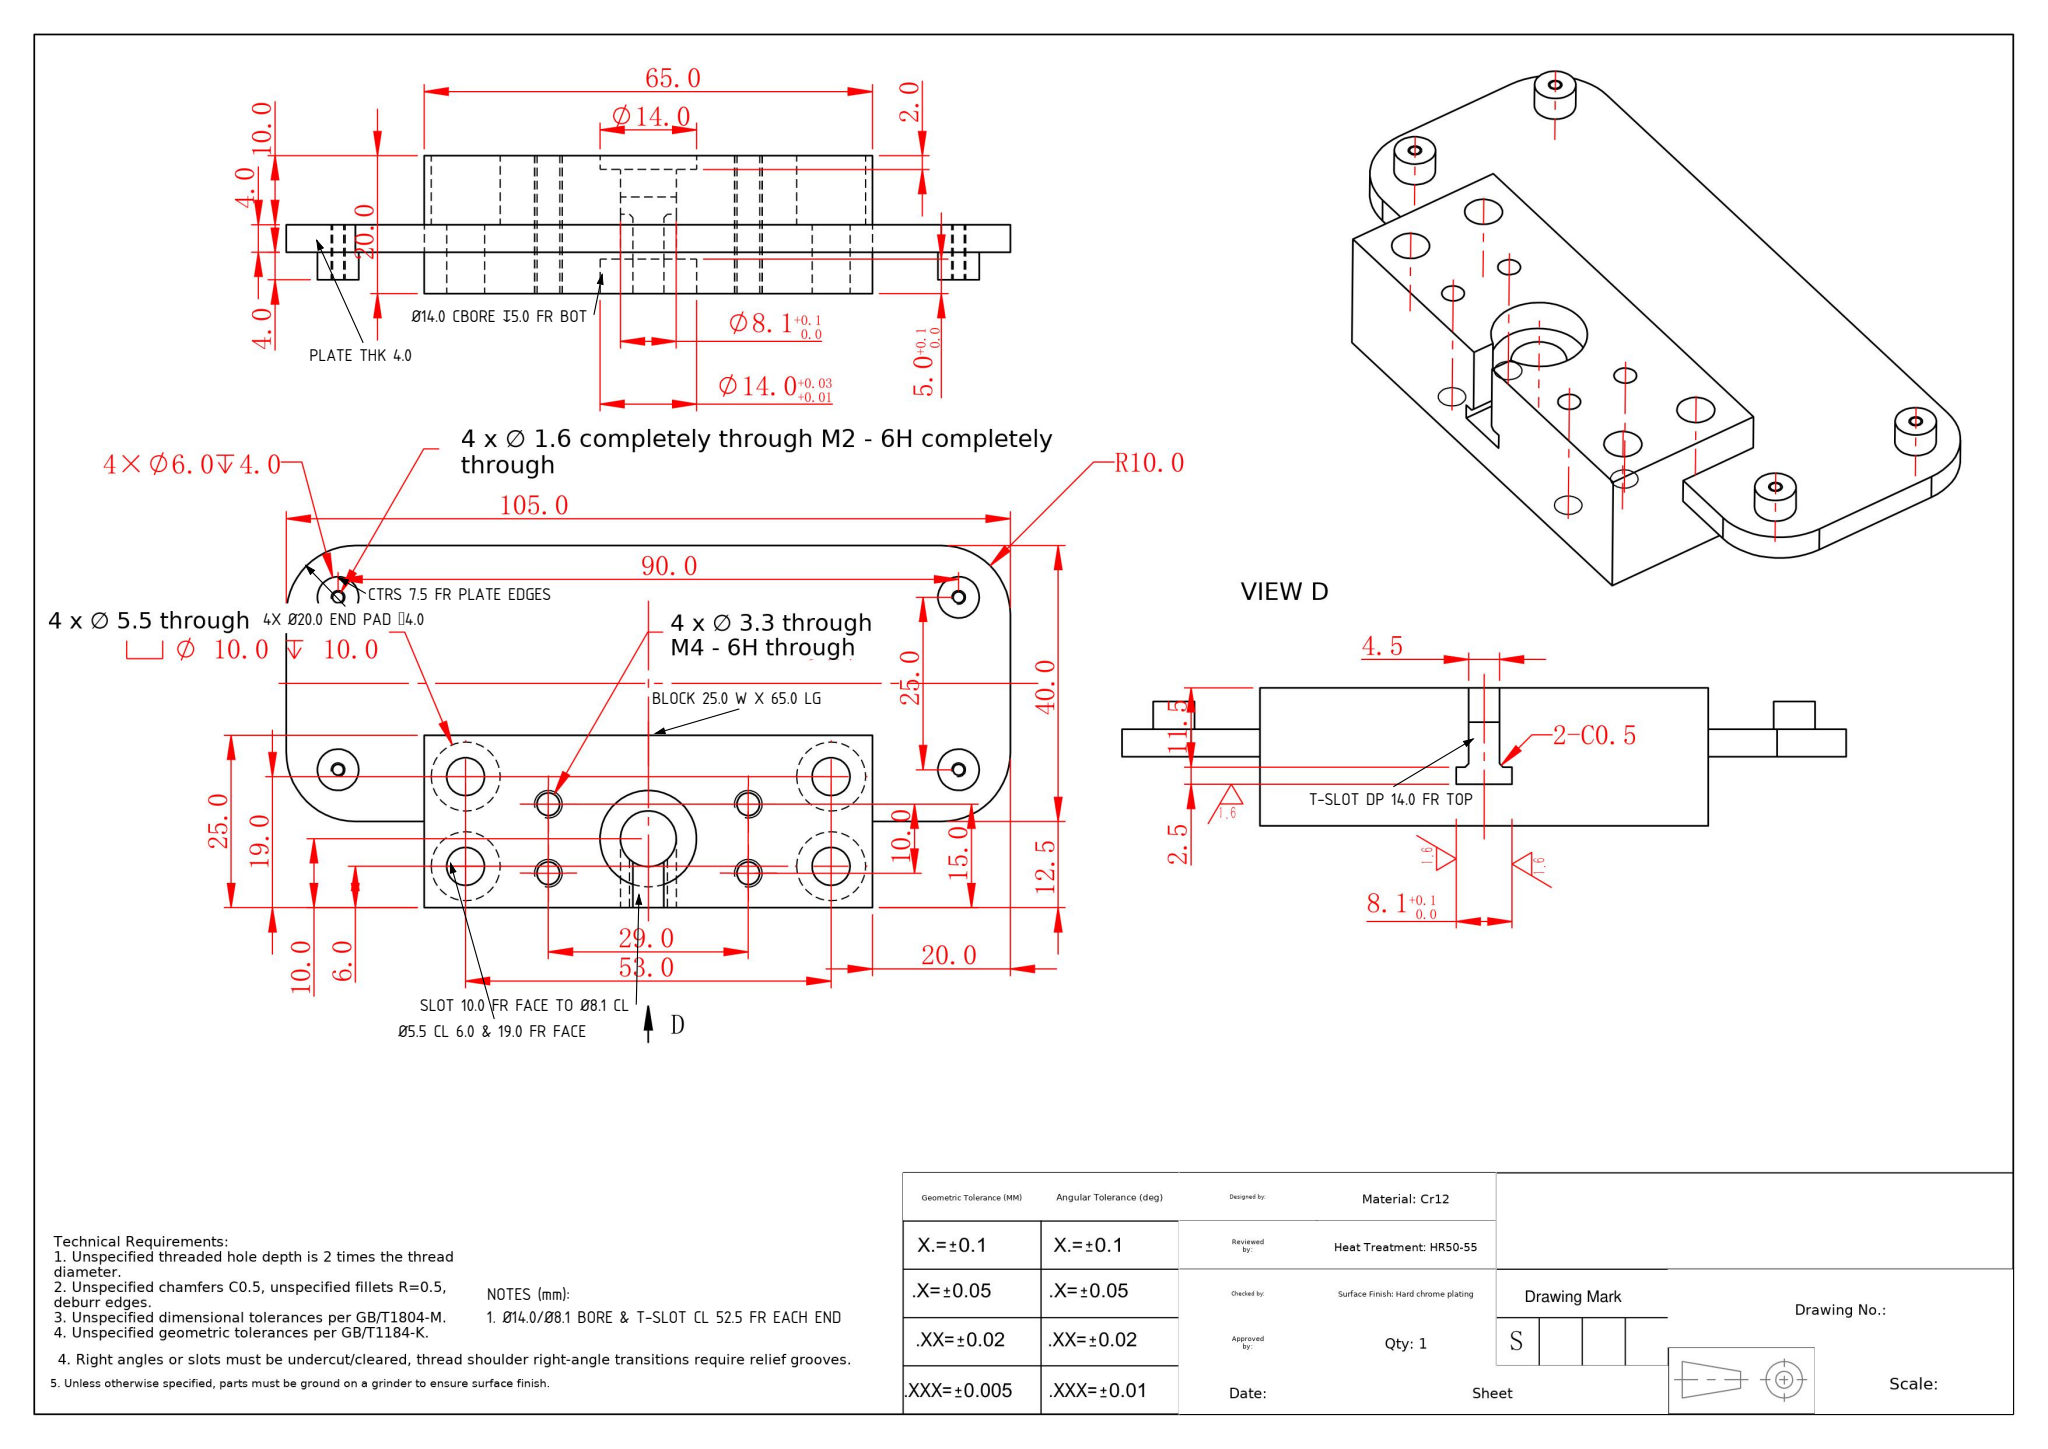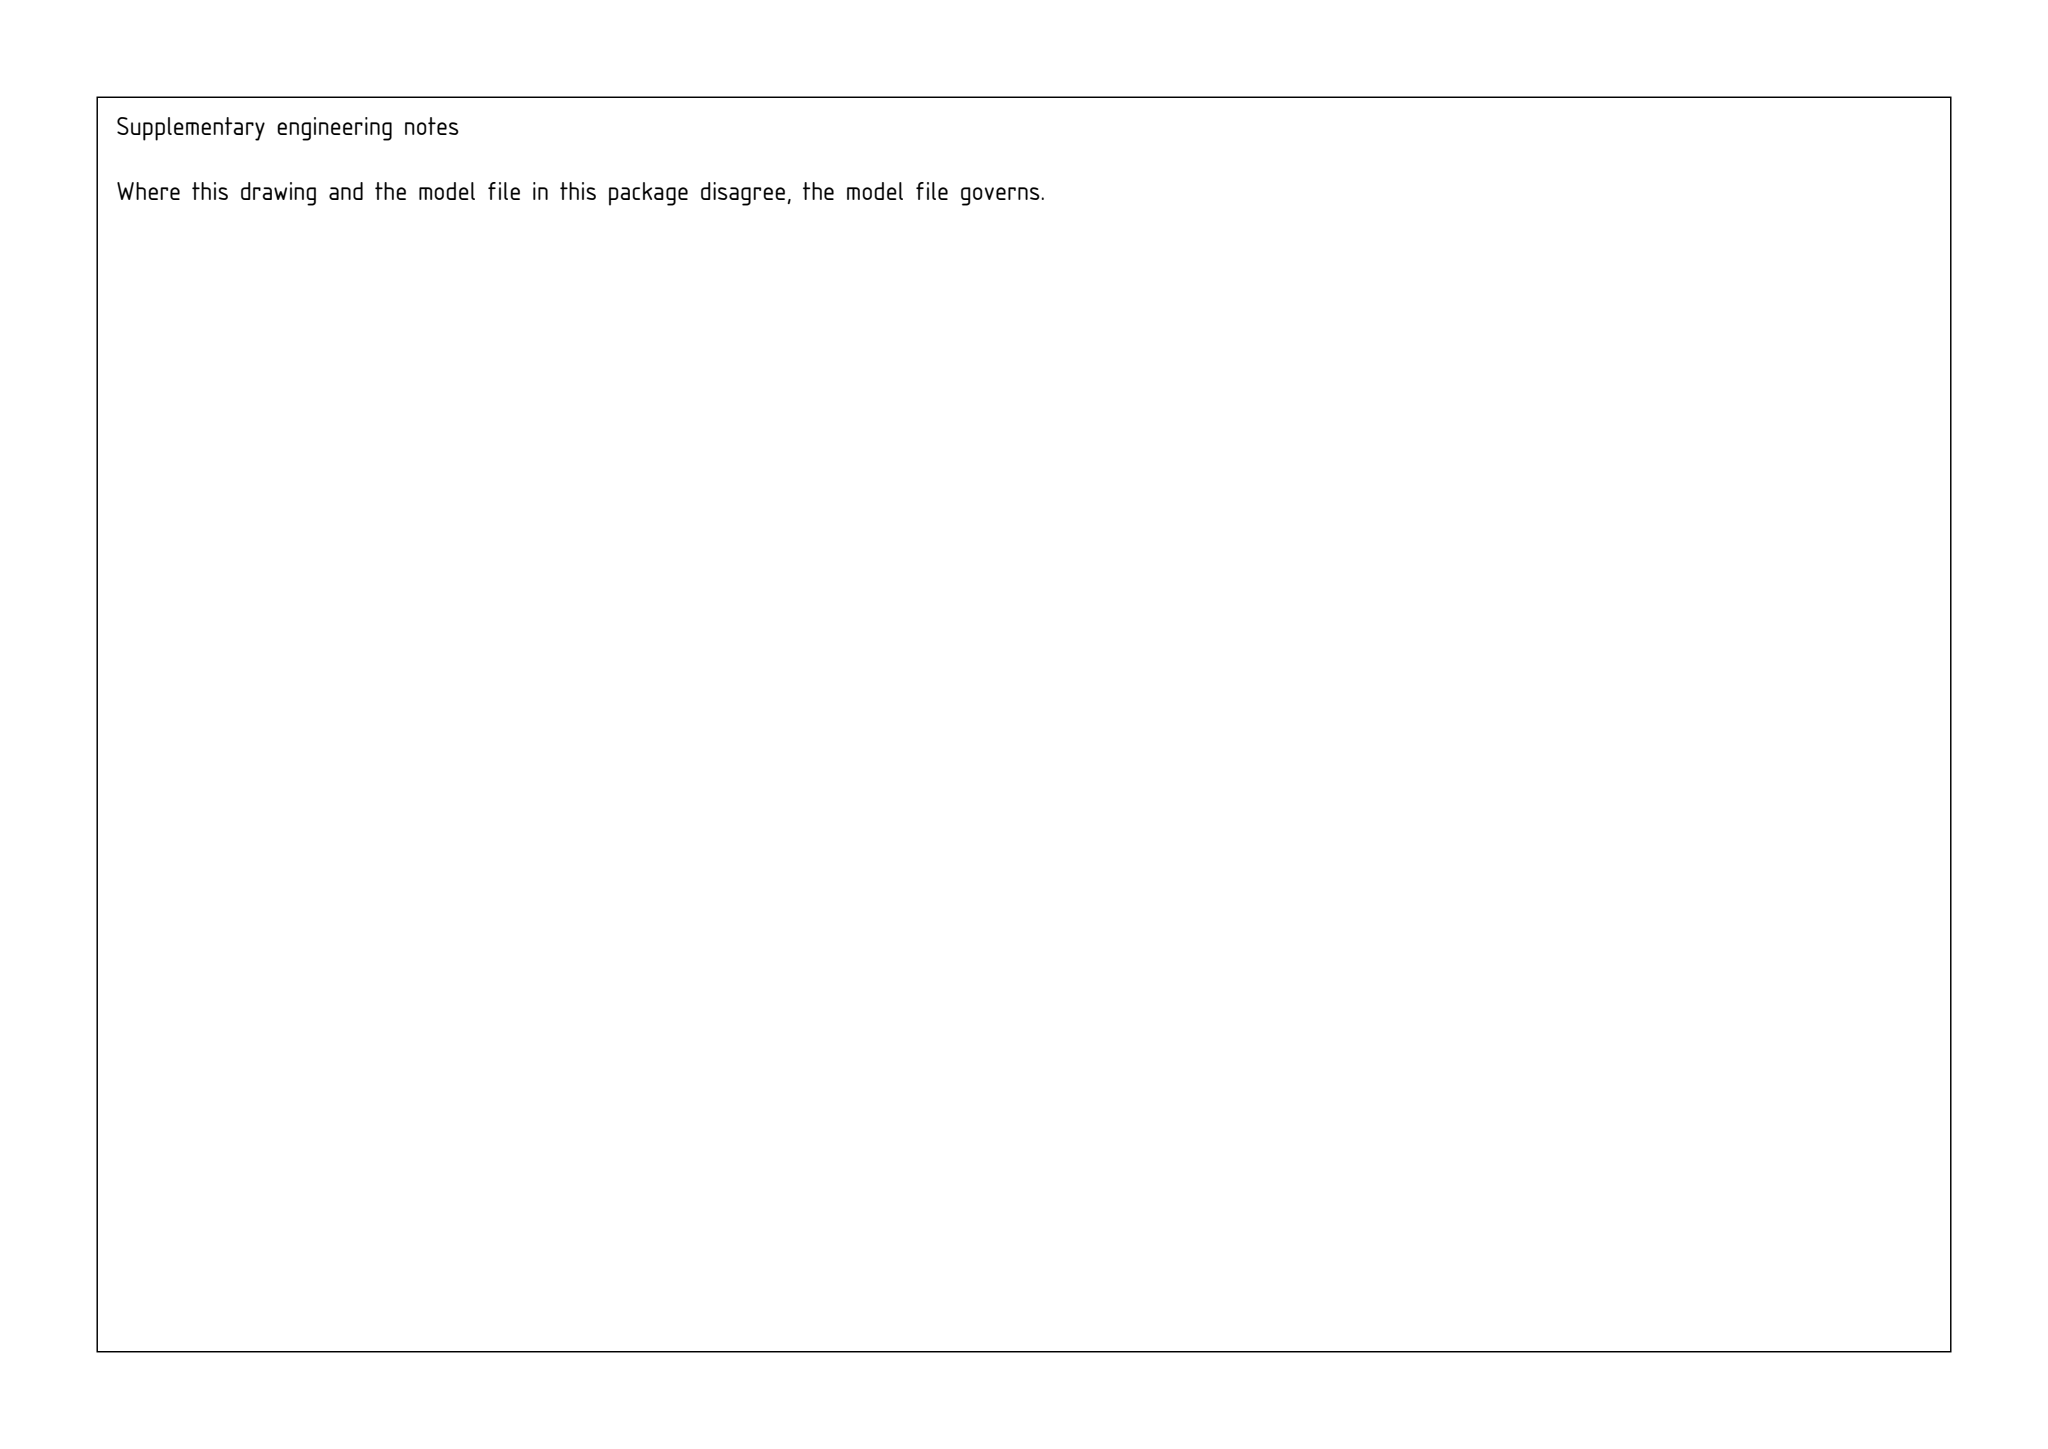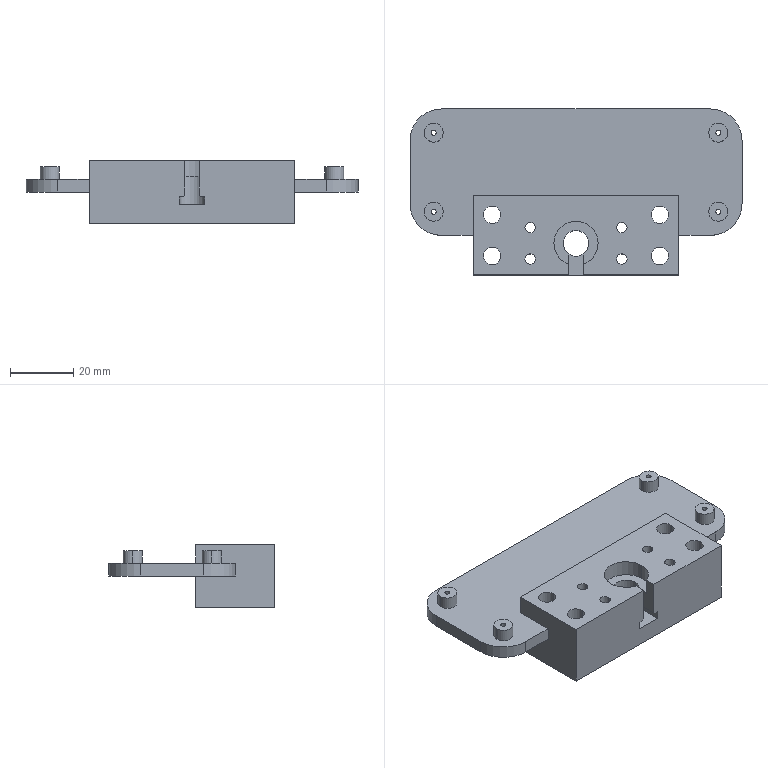Part | SolidWorks | mm | material Cr12 | 1 solid | 86 faces | box 105 x 52.5 x 20 mm | volume 39181 mm3 | cylinder 53 | plane 33 | commonest cylinder face diameters 1.6 x8 6 x8 3.3 x8 10 x8 5.5 x8 14 x5 8.1 x4 20 x4
Drawing notes:
PLATE THK 4.0, TOP FACE 6.0 BELOW BLOCK TOP FACE | from the solid: z-planes 10.0 and 14.0 bound plate; block top z=20.0 (6.0 above plate top)
RAISED BLOCK 25.0W X 65.0LG, CL 20.0 FR PLATE CL, 12.5 PAST PLATE EDGE | from the solid: block y 0-25 (CL 12.5), x 20-85; plate y 12.5-52.5 (CL 32.5), edge y=12.5
4X END PAD Ø20.0 ↑4.0 ABOVE PLATE, CTRD ON R10.0 CTRS | from the solid: cyl dia 20.0 len 4.0 at (10,22.5)(10,42.5)(95,22.5)(95,42.5), z=14 to 18
Ø14.0/Ø8.1 BORE & T-SLOT CL 52.5 FR EACH END | from the solid: bore axis at x=52.5 of 105.0 bbox; slot faces symmetric 48.45/56.55
Ø14.0 +0.03/+0.01 CBORE DP 5.0 FR BOTTOM FACE; Ø14.0 DP 2.0 FR BLOCK TOP | from the solid: Ø14 cyl len 5.0 at (52.5,10) from z=0; Ø14 cyl len 2.0 z=18.0 to 20.0 (block top)
T-SLOT NECK 4.5W DP 11.5, HEAD 8.1W X 2.5H, TOT DP 14.0 FR TOP FACE | from the solid: x planes 50.25/54.75 (4.5W) & 48.45/56.55 (8.1W); z 20.0 top, 8.5 neck btm, 6.0 slot btm
T-SLOT OPEN AT BLOCK FRONT FACE, RUNS 10.0 TO Ø8.1 BORE CL | from the solid: slot faces x=50.25/54.75 open at y=0 face, run to bore axis y=10.0
Y CL FR BLOCK FRONT FACE: Ø5.5 = 6.0 & 19.0, Ø3.3 = 5.0 & 15.0 | from the solid: Ø5.5 at y=6.0/19.0, Ø3.3 at y=5.0/15.0; block front face y=0 (block y 0-25)
4X Ø1.6/M2 & Ø6.0 DP 4.0 ON 90.0 X 25.0 CTRS, 7.5 FR PLATE EDGES | from the solid: Ø1.6/Ø6.0 at (7.5,20),(7.5,45),(97.5,20),(97.5,45); plate x 0-105, y 12.5-52.5
build123d program:
from build123d import *

# Parameters (mm, degrees)
SKETCH1_W                                          = 65
SKETCH1_H                                          = 25
BOSS_EXTRUDE1_DEPTH                                = 20
CUT_EXTRUDE1_REACH                                 = 42.156
SKETCH2_R                                          = 4.05
CUT_EXTRUDE2_REACH                                 = 47.621
CUT_EXTRUDE2_END_RADIUS                            = 4.05
SKETCH4_R                                          = 7
CUT_EXTRUDE3_DEPTH                                 = 5
CUT_EXTRUDE4_START                                 = -2
SKETCH5_R                                          = 7
CUT_EXTRUDE4_DEPTH                                 = 2
HOLE_SIZE_ACCORDING_TO_TYPE_1_OF_HEXAG_D           = 5.5
HOLE_SIZE_ACCORDING_TO_TYPE_1_OF_HEXAG_CBORE_D     = 10
HOLE_SIZE_ACCORDING_TO_TYPE_1_OF_HEXAG_CBORE_DEPTH = 10
M4_TAPPED_HOLE1_D                                  = 3.3
BOSS_EXTRUDE2_DEPTH                                = 4
FILLET1_R                                          = 10
SKETCH11_R                                         = 3
BOSS_EXTRUDE3_DEPTH                                = 4
M2_TAPPED_HOLE1_D                                  = 1.6


with BuildPart() as part:
    # Sketch1 → Boss-Extrude1 (new body)
    with BuildSketch(Plane.XY):
        Rectangle(SKETCH1_W, SKETCH1_H)
    extrude(amount=BOSS_EXTRUDE1_DEPTH)

    # Sketch2 → Cut-Extrude1 (cut, up to next)
    with BuildSketch(Plane.XY.offset(20), mode=Mode.PRIVATE) as cut_extrude1_sk1:
        with Locations((0, -2.5)):
            Circle(SKETCH2_R)
    cut_extrude1_tool1 = extrude(cut_extrude1_sk1.sketch, amount=-CUT_EXTRUDE1_REACH, mode=Mode.PRIVATE) & part.part
    add(cut_extrude1_tool1.solids().sort_by_distance((0, -2.5, 20))[0], mode=Mode.SUBTRACT)

    # Cut-Extrude2: up to this cylinder (the profile starts outside it)
    cut_extrude2_end = Plane(origin=(0, -2.5, 12.269), z_dir=(0, 0, 1)) * Cylinder(CUT_EXTRUDE2_END_RADIUS, 104.342, mode=Mode.PRIVATE)
    # Sketch3 → Cut-Extrude2 (cut, up to the surface)
    with BuildSketch(Plane.XZ.offset(12.5), mode=Mode.PRIVATE) as cut_extrude2_sk1:
        Polygon((-2.25, 20), (2.25, 20), (2.25, 9), (2.75, 8.5), (4.05, 8.5), (4.05, 6), (-4.05, 6), (-4.05, 8.5), (-2.75, 8.5), (-2.25, 9), align=None)
    cut_extrude2_tool1 = extrude(cut_extrude2_sk1.sketch, amount=-CUT_EXTRUDE2_REACH, mode=Mode.PRIVATE) - cut_extrude2_end
    add(cut_extrude2_tool1.solids().sort_by_distance((0, -12.5, 12.269))[0], mode=Mode.SUBTRACT)

    # Sketch4 → Cut-Extrude3 (cut)
    with BuildSketch(Plane.XY.offset(20)):
        with Locations((0, -2.5)):
            Circle(SKETCH4_R)
    extrude(amount=-CUT_EXTRUDE3_DEPTH, mode=Mode.SUBTRACT)

    # Sketch5 → Cut-Extrude4 (cut)
    with BuildSketch(Plane(origin=(0, 0, 0), x_dir=(-1, 0, 0), z_dir=(0, 0, -1)).offset(CUT_EXTRUDE4_START)):
        with Locations((0, -2.5)):
            Circle(SKETCH5_R)
    extrude(amount=CUT_EXTRUDE4_DEPTH, mode=Mode.SUBTRACT)

    # Hole Size _According to_ Type 1 of Hexag (through all)
    with Locations(Plane(origin=(0, 0, 0), x_dir=(-1, 0, 0), z_dir=(0, 0, -1))):
        with Locations((-26.5, 6.5), (-26.5, -6.5), (26.5, 6.5), (26.5, -6.5)):
            CounterBoreHole(HOLE_SIZE_ACCORDING_TO_TYPE_1_OF_HEXAG_D / 2, HOLE_SIZE_ACCORDING_TO_TYPE_1_OF_HEXAG_CBORE_D / 2, HOLE_SIZE_ACCORDING_TO_TYPE_1_OF_HEXAG_CBORE_DEPTH)

    # M4 Tapped Hole1 (through all)
    with Locations(Plane(origin=(0, 0, 0), x_dir=(-1, 0, 0), z_dir=(0, 0, -1))):
        with Locations((14.5, -7.5), (14.5, 2.5), (-14.5, 2.5), (-14.5, -7.5)):
            Hole(M4_TAPPED_HOLE1_D / 2)

    # Sketch10 → Boss-Extrude2 (add)
    with BuildSketch(Plane(origin=(0, 0, 10), x_dir=(-1, 0, 0), z_dir=(0, 0, -1))):
        Polygon((-32.5, 0), (-52.5, 0), (-52.5, 40), (52.5, 40), (52.5, 0), (32.5, 0), (32.5, 12.5), (-32.5, 12.5), align=None)
    extrude(amount=-BOSS_EXTRUDE2_DEPTH)

    # Fillet1
    fillet1_edges = [part.edges().sort_by_distance(p)[0] for p in [
        (52.5, 0, 12),
        (52.5, 40, 12),
        (-52.5, 40, 12),
        (-52.5, 0, 12),
    ]]
    fillet(fillet1_edges, radius=FILLET1_R)

    # Sketch11 → Boss-Extrude3 (add)
    with BuildSketch(Plane.XY.offset(14)):
        with Locations((-45, 32.5)):
            Circle(SKETCH11_R)
        with Locations((-45, 7.5)):
            Circle(SKETCH11_R)
        with Locations((45, 32.5)):
            Circle(SKETCH11_R)
        with Locations((45, 7.5)):
            Circle(SKETCH11_R)
    extrude(amount=BOSS_EXTRUDE3_DEPTH)

    # M2 Tapped Hole1 (through all)
    with Locations(Plane.XY.offset(18)):
        with Locations((-45, 32.5), (-45, 7.5), (45, 7.5), (45, 32.5)):
            Hole(M2_TAPPED_HOLE1_D / 2)


solid = part.part